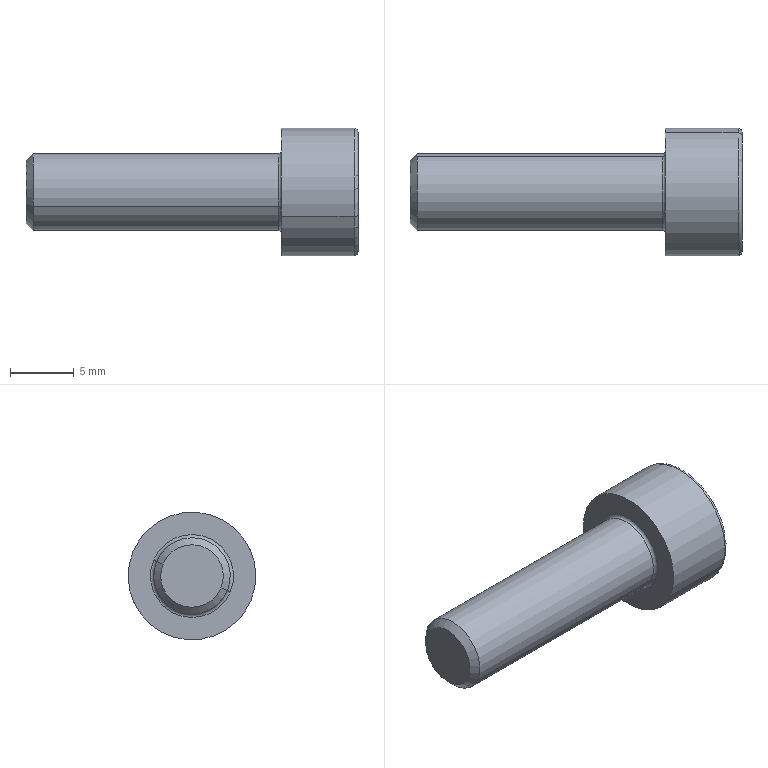Component | SolidWorks | bearing dan rumahan assembly-1_socket head cap screw_iso_M6x20-2 | 1 solid | 27 faces | box 26 x 10 x 10 mm | volume 957 mm3 | plane 15 | cone 4 | torus 4 | cylinder 4 | commonest cylinder face diameters 10 x2 6 x2
STEP:
#1=CARTESIAN_POINT('',(1.931,-4.331,3.445));
#2=VERTEX_POINT('',#1);
#3=CARTESIAN_POINT('',(1.988,-4.238,3.483));
#4=VERTEX_POINT('',#3);
#5=CARTESIAN_POINT('',(1.988,-4.238,3.483));
#6=DIRECTION('',(0.5,0.8004,0.3307));
#7=VECTOR('',#6,39.37);
#8=LINE('',#5,#7);
#9=EDGE_CURVE('',#2,#4,#8,.T.);
#10=ORIENTED_EDGE('',*,*,#9,.F.);
#11=CARTESIAN_POINT('',(1.988,-4.423,3.407));
#12=VERTEX_POINT('',#11);
#13=CARTESIAN_POINT('',(1.988,-4.423,3.407));
#14=DIRECTION('',(0.5,-0.8004,-0.3307));
#15=VECTOR('',#14,39.37);
#16=LINE('',#13,#15);
#17=EDGE_CURVE('',#2,#12,#16,.T.);
#18=ORIENTED_EDGE('',*,*,#17,.T.);
#19=CARTESIAN_POINT('',(1.988,-4.344,3.346));
#20=VERTEX_POINT('',#19);
#21=CARTESIAN_POINT('',(1.988,-4.331,3.445));
#22=DIRECTION('',(1.,0.,0.));
#23=DIRECTION('',(0.,0.9242,0.3818));
#24=AXIS2_PLACEMENT_3D('',#21,#22,#23);
#25=CIRCLE('',#24,0.0998);
#26=EDGE_CURVE('',#12,#20,#25,.T.);
#27=ORIENTED_EDGE('',*,*,#26,.T.);
#28=CARTESIAN_POINT('',(1.988,-4.252,3.384));
#29=VERTEX_POINT('',#28);
#30=CARTESIAN_POINT('',(1.988,-4.331,3.445));
#31=DIRECTION('',(1.,0.,0.));
#32=DIRECTION('',(0.,0.9242,0.3818));
#33=AXIS2_PLACEMENT_3D('',#30,#31,#32);
#34=CIRCLE('',#33,0.0998);
#35=EDGE_CURVE('',#20,#29,#34,.T.);
#36=ORIENTED_EDGE('',*,*,#35,.T.);
#37=CARTESIAN_POINT('',(1.988,-4.331,3.445));
#38=DIRECTION('',(1.,0.,0.));
#39=DIRECTION('',(0.,0.9242,0.3818));
#40=AXIS2_PLACEMENT_3D('',#37,#38,#39);
#41=CIRCLE('',#40,0.0998);
#42=EDGE_CURVE('',#29,#4,#41,.T.);
#43=ORIENTED_EDGE('',*,*,#42,.T.);
#44=EDGE_LOOP('',(#10,#18,#27,#36,#43));
#45=FACE_OUTER_BOUND('',#44,.T.);
#46=CARTESIAN_POINT('',(1.988,-4.331,3.445));
#47=DIRECTION('',(1.,0.,0.));
#48=DIRECTION('',(0.,0.9242,0.3818));
#49=AXIS2_PLACEMENT_3D('',#46,#47,#48);
#50=CONICAL_SURFACE('',#49,0.0998,1.047);
#51=ADVANCED_FACE('',(#45),#50,.F.);
#52=CARTESIAN_POINT('',(2.094,-4.513,3.37));
#53=VERTEX_POINT('',#52);
#54=CARTESIAN_POINT('',(2.094,-4.149,3.52));
#55=VERTEX_POINT('',#54);
#56=CARTESIAN_POINT('',(2.094,-4.331,3.445));
#57=DIRECTION('',(-1.,0.,0.));
#58=DIRECTION('',(0.,0.9242,0.3818));
#59=AXIS2_PLACEMENT_3D('',#56,#57,#58);
#60=CIRCLE('',#59,0.1969);
#61=EDGE_CURVE('',#53,#55,#60,.T.);
#62=ORIENTED_EDGE('',*,*,#61,.F.);
#63=CARTESIAN_POINT('',(2.106,-4.502,3.374));
#64=VERTEX_POINT('',#63);
#65=CARTESIAN_POINT('',(2.094,-4.502,3.374));
#66=DIRECTION('',(0.,-0.3818,0.9242));
#67=DIRECTION('',(0.,-0.9242,-0.3818));
#68=AXIS2_PLACEMENT_3D('',#65,#66,#67);
#69=CIRCLE('',#68,0.01181);
#70=EDGE_CURVE('',#53,#64,#69,.T.);
#71=ORIENTED_EDGE('',*,*,#70,.T.);
#72=CARTESIAN_POINT('',(2.106,-4.16,3.516));
#73=VERTEX_POINT('',#72);
#74=CARTESIAN_POINT('',(2.106,-4.331,3.445));
#75=DIRECTION('',(1.,0.,0.));
#76=DIRECTION('',(0.,0.9242,0.3818));
#77=AXIS2_PLACEMENT_3D('',#74,#75,#76);
#78=CIRCLE('',#77,0.185);
#79=EDGE_CURVE('',#73,#64,#78,.T.);
#80=ORIENTED_EDGE('',*,*,#79,.F.);
#81=CARTESIAN_POINT('',(2.094,-4.16,3.516));
#82=DIRECTION('',(0.,0.3818,-0.9242));
#83=DIRECTION('',(0.,0.9242,0.3818));
#84=AXIS2_PLACEMENT_3D('',#81,#82,#83);
#85=CIRCLE('',#84,0.01181);
#86=EDGE_CURVE('',#55,#73,#85,.T.);
#87=ORIENTED_EDGE('',*,*,#86,.F.);
#88=EDGE_LOOP('',(#62,#71,#80,#87));
#89=FACE_OUTER_BOUND('',#88,.T.);
#90=CARTESIAN_POINT('',(2.094,-4.331,3.445));
#91=DIRECTION('',(1.,0.,0.));
#92=DIRECTION('',(0.,0.9242,0.3818));
#93=AXIS2_PLACEMENT_3D('',#90,#91,#92);
#94=TOROIDAL_SURFACE('',#93,0.185,0.01181);
#95=ADVANCED_FACE('',(#89),#94,.T.);
#96=CARTESIAN_POINT('',(1.86,-4.222,3.49));
#97=VERTEX_POINT('',#96);
#98=CARTESIAN_POINT('',(1.86,-4.44,3.4));
#99=VERTEX_POINT('',#98);
#100=CARTESIAN_POINT('',(1.86,-4.331,3.445));
#101=DIRECTION('',(-1.,0.,0.));
#102=DIRECTION('',(0.,-0.9242,-0.3818));
#103=AXIS2_PLACEMENT_3D('',#100,#101,#102);
#104=CIRCLE('',#103,0.1181);
#105=EDGE_CURVE('',#97,#99,#104,.T.);
#106=ORIENTED_EDGE('',*,*,#105,.F.);
#107=CARTESIAN_POINT('',(1.87,-4.212,3.494));
#108=VERTEX_POINT('',#107);
#109=CARTESIAN_POINT('',(1.86,-4.212,3.494));
#110=DIRECTION('',(0.,-0.3818,0.9242));
#111=DIRECTION('',(0.,-0.9242,-0.3818));
#112=AXIS2_PLACEMENT_3D('',#109,#110,#111);
#113=CIRCLE('',#112,0.009843);
#114=EDGE_CURVE('',#97,#108,#113,.T.);
#115=ORIENTED_EDGE('',*,*,#114,.T.);
#116=CARTESIAN_POINT('',(1.87,-4.449,3.396));
#117=VERTEX_POINT('',#116);
#118=CARTESIAN_POINT('',(1.87,-4.331,3.445));
#119=DIRECTION('',(1.,0.,0.));
#120=DIRECTION('',(0.,-0.9242,-0.3818));
#121=AXIS2_PLACEMENT_3D('',#118,#119,#120);
#122=CIRCLE('',#121,0.128);
#123=EDGE_CURVE('',#117,#108,#122,.T.);
#124=ORIENTED_EDGE('',*,*,#123,.F.);
#125=CARTESIAN_POINT('',(1.86,-4.449,3.396));
#126=DIRECTION('',(0.,0.3818,-0.9242));
#127=DIRECTION('',(0.,0.9242,0.3818));
#128=AXIS2_PLACEMENT_3D('',#125,#126,#127);
#129=CIRCLE('',#128,0.009843);
#130=EDGE_CURVE('',#99,#117,#129,.T.);
#131=ORIENTED_EDGE('',*,*,#130,.F.);
#132=EDGE_LOOP('',(#106,#115,#124,#131));
#133=FACE_OUTER_BOUND('',#132,.T.);
#134=CARTESIAN_POINT('',(1.86,-4.331,3.445));
#135=DIRECTION('',(-1.,0.,0.));
#136=DIRECTION('',(0.,-0.9242,-0.3818));
#137=AXIS2_PLACEMENT_3D('',#134,#135,#136);
#138=TOROIDAL_SURFACE('',#137,0.128,0.009843);
#139=ADVANCED_FACE('',(#133),#138,.F.);
#140=CARTESIAN_POINT('',(1.87,-4.149,3.52));
#141=VERTEX_POINT('',#140);
#142=CARTESIAN_POINT('',(1.87,-4.513,3.37));
#143=VERTEX_POINT('',#142);
#144=CARTESIAN_POINT('',(1.87,-4.331,3.445));
#145=DIRECTION('',(1.,0.,0.));
#146=DIRECTION('',(0.,0.9242,0.3818));
#147=AXIS2_PLACEMENT_3D('',#144,#145,#146);
#148=CIRCLE('',#147,0.1969);
#149=EDGE_CURVE('',#141,#143,#148,.T.);
#150=ORIENTED_EDGE('',*,*,#149,.T.);
#151=CARTESIAN_POINT('',(3.356,-4.513,3.37));
#152=DIRECTION('',(1.,0.,0.));
#153=VECTOR('',#152,39.37);
#154=LINE('',#151,#153);
#155=EDGE_CURVE('',#143,#53,#154,.T.);
#156=ORIENTED_EDGE('',*,*,#155,.T.);
#157=ORIENTED_EDGE('',*,*,#61,.T.);
#158=CARTESIAN_POINT('',(3.356,-4.149,3.52));
#159=DIRECTION('',(1.,0.,0.));
#160=VECTOR('',#159,39.37);
#161=LINE('',#158,#160);
#162=EDGE_CURVE('',#141,#55,#161,.T.);
#163=ORIENTED_EDGE('',*,*,#162,.F.);
#164=EDGE_LOOP('',(#150,#156,#157,#163));
#165=FACE_OUTER_BOUND('',#164,.T.);
#166=CARTESIAN_POINT('',(3.356,-4.331,3.445));
#167=DIRECTION('',(1.,0.,0.));
#168=DIRECTION('',(0.,0.9242,0.3818));
#169=AXIS2_PLACEMENT_3D('',#166,#167,#168);
#170=CYLINDRICAL_SURFACE('',#169,0.1969);
#171=ADVANCED_FACE('',(#165),#170,.T.);
#172=CARTESIAN_POINT('',(1.104,-4.222,3.49));
#173=VERTEX_POINT('',#172);
#174=CARTESIAN_POINT('',(1.104,-4.44,3.4));
#175=VERTEX_POINT('',#174);
#176=CARTESIAN_POINT('',(1.104,-4.331,3.445));
#177=DIRECTION('',(1.,0.,0.));
#178=DIRECTION('',(0.,0.9242,0.3818));
#179=AXIS2_PLACEMENT_3D('',#176,#177,#178);
#180=CIRCLE('',#179,0.1181);
#181=EDGE_CURVE('',#173,#175,#180,.T.);
#182=ORIENTED_EDGE('',*,*,#181,.T.);
#183=CARTESIAN_POINT('',(3.356,-4.44,3.4));
#184=DIRECTION('',(1.,0.,0.));
#185=VECTOR('',#184,39.37);
#186=LINE('',#183,#185);
#187=EDGE_CURVE('',#175,#99,#186,.T.);
#188=ORIENTED_EDGE('',*,*,#187,.T.);
#189=CARTESIAN_POINT('',(1.86,-4.331,3.445));
#190=DIRECTION('',(-1.,0.,0.));
#191=DIRECTION('',(0.,-0.9242,-0.3818));
#192=AXIS2_PLACEMENT_3D('',#189,#190,#191);
#193=CIRCLE('',#192,0.1181);
#194=EDGE_CURVE('',#99,#97,#193,.T.);
#195=ORIENTED_EDGE('',*,*,#194,.T.);
#196=CARTESIAN_POINT('',(3.356,-4.222,3.49));
#197=DIRECTION('',(1.,0.,0.));
#198=VECTOR('',#197,39.37);
#199=LINE('',#196,#198);
#200=EDGE_CURVE('',#173,#97,#199,.T.);
#201=ORIENTED_EDGE('',*,*,#200,.F.);
#202=EDGE_LOOP('',(#182,#188,#195,#201));
#203=FACE_OUTER_BOUND('',#202,.T.);
#204=CARTESIAN_POINT('',(3.356,-4.331,3.445));
#205=DIRECTION('',(1.,0.,0.));
#206=DIRECTION('',(0.,0.9242,0.3818));
#207=AXIS2_PLACEMENT_3D('',#204,#205,#206);
#208=CYLINDRICAL_SURFACE('',#207,0.1181);
#209=ADVANCED_FACE('',(#203),#208,.T.);
#210=CARTESIAN_POINT('',(1.083,-4.242,3.482));
#211=VERTEX_POINT('',#210);
#212=CARTESIAN_POINT('',(1.083,-4.42,3.408));
#213=VERTEX_POINT('',#212);
#214=CARTESIAN_POINT('',(1.083,-4.331,3.445));
#215=DIRECTION('',(1.,0.,0.));
#216=DIRECTION('',(0.,0.9242,0.3818));
#217=AXIS2_PLACEMENT_3D('',#214,#215,#216);
#218=CIRCLE('',#217,0.0965);
#219=EDGE_CURVE('',#211,#213,#218,.T.);
#220=ORIENTED_EDGE('',*,*,#219,.T.);
#221=CARTESIAN_POINT('',(1.083,-4.42,3.408));
#222=DIRECTION('',(0.7071,-0.6535,-0.27));
#223=VECTOR('',#222,39.37);
#224=LINE('',#221,#223);
#225=EDGE_CURVE('',#213,#175,#224,.T.);
#226=ORIENTED_EDGE('',*,*,#225,.T.);
#227=ORIENTED_EDGE('',*,*,#181,.F.);
#228=CARTESIAN_POINT('',(1.083,-4.242,3.482));
#229=DIRECTION('',(0.7071,0.6535,0.27));
#230=VECTOR('',#229,39.37);
#231=LINE('',#228,#230);
#232=EDGE_CURVE('',#211,#173,#231,.T.);
#233=ORIENTED_EDGE('',*,*,#232,.F.);
#234=EDGE_LOOP('',(#220,#226,#227,#233));
#235=FACE_OUTER_BOUND('',#234,.T.);
#236=CARTESIAN_POINT('',(1.083,-4.331,3.445));
#237=DIRECTION('',(1.,0.,0.));
#238=DIRECTION('',(0.,0.9242,0.3818));
#239=AXIS2_PLACEMENT_3D('',#236,#237,#238);
#240=CONICAL_SURFACE('',#239,0.0965,0.7854);
#241=ADVANCED_FACE('',(#235),#240,.T.);
#242=CARTESIAN_POINT('',(2.106,-4.375,3.551));
#243=VERTEX_POINT('',#242);
#244=CARTESIAN_POINT('',(2.106,-4.26,3.536));
#245=VERTEX_POINT('',#244);
#246=CARTESIAN_POINT('',(2.106,-4.375,3.551));
#247=DIRECTION('',(0.,0.9913,-0.1314));
#248=VECTOR('',#247,39.37);
#249=LINE('',#246,#248);
#250=EDGE_CURVE('',#243,#245,#249,.T.);
#251=ORIENTED_EDGE('',*,*,#250,.T.);
#252=CARTESIAN_POINT('',(2.106,-4.216,3.43));
#253=VERTEX_POINT('',#252);
#254=CARTESIAN_POINT('',(2.106,-4.216,3.43));
#255=DIRECTION('',(0.,-0.3818,0.9242));
#256=VECTOR('',#255,39.37);
#257=LINE('',#254,#256);
#258=EDGE_CURVE('',#253,#245,#257,.T.);
#259=ORIENTED_EDGE('',*,*,#258,.F.);
#260=CARTESIAN_POINT('',(2.106,-4.287,3.338));
#261=VERTEX_POINT('',#260);
#262=CARTESIAN_POINT('',(2.106,-4.216,3.43));
#263=DIRECTION('',(0.,-0.6095,-0.7928));
#264=VECTOR('',#263,39.37);
#265=LINE('',#262,#264);
#266=EDGE_CURVE('',#253,#261,#265,.T.);
#267=ORIENTED_EDGE('',*,*,#266,.T.);
#268=CARTESIAN_POINT('',(2.106,-4.401,3.354));
#269=VERTEX_POINT('',#268);
#270=CARTESIAN_POINT('',(2.106,-4.287,3.338));
#271=DIRECTION('',(0.,-0.9913,0.1314));
#272=VECTOR('',#271,39.37);
#273=LINE('',#270,#272);
#274=EDGE_CURVE('',#261,#269,#273,.T.);
#275=ORIENTED_EDGE('',*,*,#274,.T.);
#276=CARTESIAN_POINT('',(2.106,-4.445,3.46));
#277=VERTEX_POINT('',#276);
#278=CARTESIAN_POINT('',(2.106,-4.445,3.46));
#279=DIRECTION('',(0.,0.3818,-0.9242));
#280=VECTOR('',#279,39.37);
#281=LINE('',#278,#280);
#282=EDGE_CURVE('',#277,#269,#281,.T.);
#283=ORIENTED_EDGE('',*,*,#282,.F.);
#284=CARTESIAN_POINT('',(2.106,-4.375,3.551));
#285=DIRECTION('',(0.,-0.6095,-0.7928));
#286=VECTOR('',#285,39.37);
#287=LINE('',#284,#286);
#288=EDGE_CURVE('',#243,#277,#287,.T.);
#289=ORIENTED_EDGE('',*,*,#288,.F.);
#290=EDGE_LOOP('',(#251,#259,#267,#275,#283,#289));
#291=FACE_BOUND('',#290,.T.);
#292=ORIENTED_EDGE('',*,*,#79,.T.);
#293=CARTESIAN_POINT('',(2.106,-4.331,3.445));
#294=DIRECTION('',(1.,0.,0.));
#295=DIRECTION('',(0.,0.9242,0.3818));
#296=AXIS2_PLACEMENT_3D('',#293,#294,#295);
#297=CIRCLE('',#296,0.185);
#298=EDGE_CURVE('',#64,#73,#297,.T.);
#299=ORIENTED_EDGE('',*,*,#298,.T.);
#300=EDGE_LOOP('',(#292,#299));
#301=FACE_OUTER_BOUND('',#300,.T.);
#302=CARTESIAN_POINT('',(2.106,-4.331,3.445));
#303=DIRECTION('',(1.,0.,0.));
#304=DIRECTION('',(0.,0.9242,0.3818));
#305=AXIS2_PLACEMENT_3D('',#302,#303,#304);
#306=PLANE('',#305);
#307=ADVANCED_FACE('',(#291,#301),#306,.T.);
#308=ORIENTED_EDGE('',*,*,#219,.F.);
#309=CARTESIAN_POINT('',(1.083,-4.331,3.445));
#310=DIRECTION('',(1.,0.,0.));
#311=DIRECTION('',(0.,0.9242,0.3818));
#312=AXIS2_PLACEMENT_3D('',#309,#310,#311);
#313=CIRCLE('',#312,0.0965);
#314=EDGE_CURVE('',#213,#211,#313,.T.);
#315=ORIENTED_EDGE('',*,*,#314,.F.);
#316=EDGE_LOOP('',(#308,#315));
#317=FACE_OUTER_BOUND('',#316,.T.);
#318=CARTESIAN_POINT('',(1.083,-4.368,3.534));
#319=DIRECTION('',(-1.,0.,0.));
#320=DIRECTION('',(0.,-0.9242,-0.3818));
#321=AXIS2_PLACEMENT_3D('',#318,#319,#320);
#322=PLANE('',#321);
#323=ADVANCED_FACE('',(#317),#322,.T.);
#324=ORIENTED_EDGE('',*,*,#225,.F.);
#325=ORIENTED_EDGE('',*,*,#314,.T.);
#326=ORIENTED_EDGE('',*,*,#232,.T.);
#327=CARTESIAN_POINT('',(1.104,-4.331,3.445));
#328=DIRECTION('',(1.,0.,0.));
#329=DIRECTION('',(0.,0.9242,0.3818));
#330=AXIS2_PLACEMENT_3D('',#327,#328,#329);
#331=CIRCLE('',#330,0.1181);
#332=EDGE_CURVE('',#175,#173,#331,.T.);
#333=ORIENTED_EDGE('',*,*,#332,.F.);
#334=EDGE_LOOP('',(#324,#325,#326,#333));
#335=FACE_OUTER_BOUND('',#334,.T.);
#336=CARTESIAN_POINT('',(1.083,-4.331,3.445));
#337=DIRECTION('',(1.,0.,0.));
#338=DIRECTION('',(0.,0.9242,0.3818));
#339=AXIS2_PLACEMENT_3D('',#336,#337,#338);
#340=CONICAL_SURFACE('',#339,0.0965,0.7854);
#341=ADVANCED_FACE('',(#335),#340,.T.);
#342=ORIENTED_EDGE('',*,*,#187,.F.);
#343=ORIENTED_EDGE('',*,*,#332,.T.);
#344=ORIENTED_EDGE('',*,*,#200,.T.);
#345=ORIENTED_EDGE('',*,*,#105,.T.);
#346=EDGE_LOOP('',(#342,#343,#344,#345));
#347=FACE_OUTER_BOUND('',#346,.T.);
#348=CARTESIAN_POINT('',(3.356,-4.331,3.445));
#349=DIRECTION('',(1.,0.,0.));
#350=DIRECTION('',(0.,0.9242,0.3818));
#351=AXIS2_PLACEMENT_3D('',#348,#349,#350);
#352=CYLINDRICAL_SURFACE('',#351,0.1181);
#353=ADVANCED_FACE('',(#347),#352,.T.);
#354=ORIENTED_EDGE('',*,*,#123,.T.);
#355=CARTESIAN_POINT('',(1.87,-4.331,3.445));
#356=DIRECTION('',(1.,0.,0.));
#357=DIRECTION('',(0.,-0.9242,-0.3818));
#358=AXIS2_PLACEMENT_3D('',#355,#356,#357);
#359=CIRCLE('',#358,0.128);
#360=EDGE_CURVE('',#108,#117,#359,.T.);
#361=ORIENTED_EDGE('',*,*,#360,.T.);
#362=EDGE_LOOP('',(#354,#361));
#363=FACE_BOUND('',#362,.T.);
#364=ORIENTED_EDGE('',*,*,#149,.F.);
#365=CARTESIAN_POINT('',(1.87,-4.331,3.445));
#366=DIRECTION('',(1.,0.,0.));
#367=DIRECTION('',(0.,0.9242,0.3818));
#368=AXIS2_PLACEMENT_3D('',#365,#366,#367);
#369=CIRCLE('',#368,0.1969);
#370=EDGE_CURVE('',#143,#141,#369,.T.);
#371=ORIENTED_EDGE('',*,*,#370,.F.);
#372=EDGE_LOOP('',(#364,#371));
#373=FACE_OUTER_BOUND('',#372,.T.);
#374=CARTESIAN_POINT('',(1.87,-4.406,3.627));
#375=DIRECTION('',(-1.,0.,0.));
#376=DIRECTION('',(0.,-0.9242,-0.3818));
#377=AXIS2_PLACEMENT_3D('',#374,#375,#376);
#378=PLANE('',#377);
#379=ADVANCED_FACE('',(#363,#373),#378,.T.);
#380=ORIENTED_EDGE('',*,*,#155,.F.);
#381=ORIENTED_EDGE('',*,*,#370,.T.);
#382=ORIENTED_EDGE('',*,*,#162,.T.);
#383=CARTESIAN_POINT('',(2.094,-4.331,3.445));
#384=DIRECTION('',(-1.,0.,0.));
#385=DIRECTION('',(0.,0.9242,0.3818));
#386=AXIS2_PLACEMENT_3D('',#383,#384,#385);
#387=CIRCLE('',#386,0.1969);
#388=EDGE_CURVE('',#55,#53,#387,.T.);
#389=ORIENTED_EDGE('',*,*,#388,.T.);
#390=EDGE_LOOP('',(#380,#381,#382,#389));
#391=FACE_OUTER_BOUND('',#390,.T.);
#392=CARTESIAN_POINT('',(3.356,-4.331,3.445));
#393=DIRECTION('',(1.,0.,0.));
#394=DIRECTION('',(0.,0.9242,0.3818));
#395=AXIS2_PLACEMENT_3D('',#392,#393,#394);
#396=CYLINDRICAL_SURFACE('',#395,0.1969);
#397=ADVANCED_FACE('',(#391),#396,.T.);
#398=ORIENTED_EDGE('',*,*,#114,.F.);
#399=ORIENTED_EDGE('',*,*,#194,.F.);
#400=ORIENTED_EDGE('',*,*,#130,.T.);
#401=ORIENTED_EDGE('',*,*,#360,.F.);
#402=EDGE_LOOP('',(#398,#399,#400,#401));
#403=FACE_OUTER_BOUND('',#402,.T.);
#404=CARTESIAN_POINT('',(1.86,-4.331,3.445));
#405=DIRECTION('',(-1.,0.,0.));
#406=DIRECTION('',(0.,-0.9242,-0.3818));
#407=AXIS2_PLACEMENT_3D('',#404,#405,#406);
#408=TOROIDAL_SURFACE('',#407,0.128,0.009843);
#409=ADVANCED_FACE('',(#403),#408,.F.);
#410=ORIENTED_EDGE('',*,*,#70,.F.);
#411=ORIENTED_EDGE('',*,*,#388,.F.);
#412=ORIENTED_EDGE('',*,*,#86,.T.);
#413=ORIENTED_EDGE('',*,*,#298,.F.);
#414=EDGE_LOOP('',(#410,#411,#412,#413));
#415=FACE_OUTER_BOUND('',#414,.T.);
#416=CARTESIAN_POINT('',(2.094,-4.331,3.445));
#417=DIRECTION('',(1.,0.,0.));
#418=DIRECTION('',(0.,0.9242,0.3818));
#419=AXIS2_PLACEMENT_3D('',#416,#417,#418);
#420=TOROIDAL_SURFACE('',#419,0.185,0.01181);
#421=ADVANCED_FACE('',(#415),#420,.T.);
#422=ORIENTED_EDGE('',*,*,#250,.F.);
#423=CARTESIAN_POINT('',(1.988,-4.375,3.551));
#424=VERTEX_POINT('',#423);
#425=CARTESIAN_POINT('',(1.988,-4.375,3.551));
#426=DIRECTION('',(1.,0.,0.));
#427=VECTOR('',#426,39.37);
#428=LINE('',#425,#427);
#429=EDGE_CURVE('',#424,#243,#428,.T.);
#430=ORIENTED_EDGE('',*,*,#429,.F.);
#431=CARTESIAN_POINT('',(1.988,-4.318,3.544));
#432=VERTEX_POINT('',#431);
#433=CARTESIAN_POINT('',(1.988,-4.375,3.551));
#434=DIRECTION('',(0.,0.9913,-0.1314));
#435=VECTOR('',#434,39.37);
#436=LINE('',#433,#435);
#437=EDGE_CURVE('',#424,#432,#436,.T.);
#438=ORIENTED_EDGE('',*,*,#437,.T.);
#439=CARTESIAN_POINT('',(1.988,-4.26,3.536));
#440=VERTEX_POINT('',#439);
#441=CARTESIAN_POINT('',(1.988,-4.375,3.551));
#442=DIRECTION('',(0.,0.9913,-0.1314));
#443=VECTOR('',#442,39.37);
#444=LINE('',#441,#443);
#445=EDGE_CURVE('',#432,#440,#444,.T.);
#446=ORIENTED_EDGE('',*,*,#445,.T.);
#447=CARTESIAN_POINT('',(1.988,-4.26,3.536));
#448=DIRECTION('',(1.,0.,0.));
#449=VECTOR('',#448,39.37);
#450=LINE('',#447,#449);
#451=EDGE_CURVE('',#440,#245,#450,.T.);
#452=ORIENTED_EDGE('',*,*,#451,.T.);
#453=EDGE_LOOP('',(#422,#430,#438,#446,#452));
#454=FACE_OUTER_BOUND('',#453,.T.);
#455=CARTESIAN_POINT('',(1.988,-4.375,3.551));
#456=DIRECTION('',(0.,-0.1314,-0.9913));
#457=DIRECTION('',(0.,-0.9913,0.1314));
#458=AXIS2_PLACEMENT_3D('',#455,#456,#457);
#459=PLANE('',#458);
#460=ADVANCED_FACE('',(#454),#459,.T.);
#461=ORIENTED_EDGE('',*,*,#258,.T.);
#462=ORIENTED_EDGE('',*,*,#451,.F.);
#463=CARTESIAN_POINT('',(1.988,-4.216,3.43));
#464=DIRECTION('',(0.,-0.3818,0.9242));
#465=VECTOR('',#464,39.37);
#466=LINE('',#463,#465);
#467=EDGE_CURVE('',#4,#440,#466,.T.);
#468=ORIENTED_EDGE('',*,*,#467,.F.);
#469=CARTESIAN_POINT('',(1.988,-4.216,3.43));
#470=VERTEX_POINT('',#469);
#471=CARTESIAN_POINT('',(1.988,-4.216,3.43));
#472=DIRECTION('',(0.,-0.3818,0.9242));
#473=VECTOR('',#472,39.37);
#474=LINE('',#471,#473);
#475=EDGE_CURVE('',#470,#4,#474,.T.);
#476=ORIENTED_EDGE('',*,*,#475,.F.);
#477=CARTESIAN_POINT('',(1.988,-4.216,3.43));
#478=DIRECTION('',(1.,0.,0.));
#479=VECTOR('',#478,39.37);
#480=LINE('',#477,#479);
#481=EDGE_CURVE('',#470,#253,#480,.T.);
#482=ORIENTED_EDGE('',*,*,#481,.T.);
#483=EDGE_LOOP('',(#461,#462,#468,#476,#482));
#484=FACE_OUTER_BOUND('',#483,.T.);
#485=CARTESIAN_POINT('',(1.988,-4.216,3.43));
#486=DIRECTION('',(0.,0.9242,0.3818));
#487=DIRECTION('',(0.,0.3818,-0.9242));
#488=AXIS2_PLACEMENT_3D('',#485,#486,#487);
#489=PLANE('',#488);
#490=ADVANCED_FACE('',(#484),#489,.F.);
#491=ORIENTED_EDGE('',*,*,#266,.F.);
#492=ORIENTED_EDGE('',*,*,#481,.F.);
#493=CARTESIAN_POINT('',(1.988,-4.216,3.43));
#494=DIRECTION('',(0.,-0.6095,-0.7928));
#495=VECTOR('',#494,39.37);
#496=LINE('',#493,#495);
#497=EDGE_CURVE('',#470,#29,#496,.T.);
#498=ORIENTED_EDGE('',*,*,#497,.T.);
#499=CARTESIAN_POINT('',(1.988,-4.287,3.338));
#500=VERTEX_POINT('',#499);
#501=CARTESIAN_POINT('',(1.988,-4.216,3.43));
#502=DIRECTION('',(0.,-0.6095,-0.7928));
#503=VECTOR('',#502,39.37);
#504=LINE('',#501,#503);
#505=EDGE_CURVE('',#29,#500,#504,.T.);
#506=ORIENTED_EDGE('',*,*,#505,.T.);
#507=CARTESIAN_POINT('',(1.988,-4.287,3.338));
#508=DIRECTION('',(1.,0.,0.));
#509=VECTOR('',#508,39.37);
#510=LINE('',#507,#509);
#511=EDGE_CURVE('',#500,#261,#510,.T.);
#512=ORIENTED_EDGE('',*,*,#511,.T.);
#513=EDGE_LOOP('',(#491,#492,#498,#506,#512));
#514=FACE_OUTER_BOUND('',#513,.T.);
#515=CARTESIAN_POINT('',(1.988,-4.216,3.43));
#516=DIRECTION('',(0.,-0.7928,0.6095));
#517=DIRECTION('',(0.,0.6095,0.7928));
#518=AXIS2_PLACEMENT_3D('',#515,#516,#517);
#519=PLANE('',#518);
#520=ADVANCED_FACE('',(#514),#519,.T.);
#521=ORIENTED_EDGE('',*,*,#274,.F.);
#522=ORIENTED_EDGE('',*,*,#511,.F.);
#523=CARTESIAN_POINT('',(1.988,-4.287,3.338));
#524=DIRECTION('',(0.,-0.9913,0.1314));
#525=VECTOR('',#524,39.37);
#526=LINE('',#523,#525);
#527=EDGE_CURVE('',#500,#20,#526,.T.);
#528=ORIENTED_EDGE('',*,*,#527,.T.);
#529=CARTESIAN_POINT('',(1.988,-4.401,3.354));
#530=VERTEX_POINT('',#529);
#531=CARTESIAN_POINT('',(1.988,-4.287,3.338));
#532=DIRECTION('',(0.,-0.9913,0.1314));
#533=VECTOR('',#532,39.37);
#534=LINE('',#531,#533);
#535=EDGE_CURVE('',#20,#530,#534,.T.);
#536=ORIENTED_EDGE('',*,*,#535,.T.);
#537=CARTESIAN_POINT('',(1.988,-4.401,3.354));
#538=DIRECTION('',(1.,0.,0.));
#539=VECTOR('',#538,39.37);
#540=LINE('',#537,#539);
#541=EDGE_CURVE('',#530,#269,#540,.T.);
#542=ORIENTED_EDGE('',*,*,#541,.T.);
#543=EDGE_LOOP('',(#521,#522,#528,#536,#542));
#544=FACE_OUTER_BOUND('',#543,.T.);
#545=CARTESIAN_POINT('',(1.988,-4.287,3.338));
#546=DIRECTION('',(0.,0.1314,0.9913));
#547=DIRECTION('',(0.,0.9913,-0.1314));
#548=AXIS2_PLACEMENT_3D('',#545,#546,#547);
#549=PLANE('',#548);
#550=ADVANCED_FACE('',(#544),#549,.T.);
#551=ORIENTED_EDGE('',*,*,#282,.T.);
#552=ORIENTED_EDGE('',*,*,#541,.F.);
#553=CARTESIAN_POINT('',(1.988,-4.445,3.46));
#554=DIRECTION('',(0.,0.3818,-0.9242));
#555=VECTOR('',#554,39.37);
#556=LINE('',#553,#555);
#557=EDGE_CURVE('',#12,#530,#556,.T.);
#558=ORIENTED_EDGE('',*,*,#557,.F.);
#559=CARTESIAN_POINT('',(1.988,-4.445,3.46));
#560=VERTEX_POINT('',#559);
#561=CARTESIAN_POINT('',(1.988,-4.445,3.46));
#562=DIRECTION('',(0.,0.3818,-0.9242));
#563=VECTOR('',#562,39.37);
#564=LINE('',#561,#563);
#565=EDGE_CURVE('',#560,#12,#564,.T.);
#566=ORIENTED_EDGE('',*,*,#565,.F.);
#567=CARTESIAN_POINT('',(1.988,-4.445,3.46));
#568=DIRECTION('',(1.,0.,0.));
#569=VECTOR('',#568,39.37);
#570=LINE('',#567,#569);
#571=EDGE_CURVE('',#560,#277,#570,.T.);
#572=ORIENTED_EDGE('',*,*,#571,.T.);
#573=EDGE_LOOP('',(#551,#552,#558,#566,#572));
#574=FACE_OUTER_BOUND('',#573,.T.);
#575=CARTESIAN_POINT('',(1.988,-4.445,3.46));
#576=DIRECTION('',(0.,-0.9242,-0.3818));
#577=DIRECTION('',(0.,-0.3818,0.9242));
#578=AXIS2_PLACEMENT_3D('',#575,#576,#577);
#579=PLANE('',#578);
#580=ADVANCED_FACE('',(#574),#579,.F.);
#581=ORIENTED_EDGE('',*,*,#288,.T.);
#582=ORIENTED_EDGE('',*,*,#571,.F.);
#583=CARTESIAN_POINT('',(1.988,-4.41,3.506));
#584=VERTEX_POINT('',#583);
#585=CARTESIAN_POINT('',(1.988,-4.375,3.551));
#586=DIRECTION('',(0.,-0.6095,-0.7928));
#587=VECTOR('',#586,39.37);
#588=LINE('',#585,#587);
#589=EDGE_CURVE('',#584,#560,#588,.T.);
#590=ORIENTED_EDGE('',*,*,#589,.F.);
#591=CARTESIAN_POINT('',(1.988,-4.375,3.551));
#592=DIRECTION('',(0.,-0.6095,-0.7928));
#593=VECTOR('',#592,39.37);
#594=LINE('',#591,#593);
#595=EDGE_CURVE('',#424,#584,#594,.T.);
#596=ORIENTED_EDGE('',*,*,#595,.F.);
#597=ORIENTED_EDGE('',*,*,#429,.T.);
#598=EDGE_LOOP('',(#581,#582,#590,#596,#597));
#599=FACE_OUTER_BOUND('',#598,.T.);
#600=CARTESIAN_POINT('',(1.988,-4.375,3.551));
#601=DIRECTION('',(0.,-0.7928,0.6095));
#602=DIRECTION('',(0.,0.6095,0.7928));
#603=AXIS2_PLACEMENT_3D('',#600,#601,#602);
#604=PLANE('',#603);
#605=ADVANCED_FACE('',(#599),#604,.F.);
#606=ORIENTED_EDGE('',*,*,#557,.T.);
#607=ORIENTED_EDGE('',*,*,#535,.F.);
#608=ORIENTED_EDGE('',*,*,#26,.F.);
#609=EDGE_LOOP('',(#606,#607,#608));
#610=FACE_OUTER_BOUND('',#609,.T.);
#611=CARTESIAN_POINT('',(1.988,-4.375,3.551));
#612=DIRECTION('',(-1.,0.,0.));
#613=DIRECTION('',(0.,-0.9242,-0.3818));
#614=AXIS2_PLACEMENT_3D('',#611,#612,#613);
#615=PLANE('',#614);
#616=ADVANCED_FACE('',(#610),#615,.F.);
#617=ORIENTED_EDGE('',*,*,#527,.F.);
#618=ORIENTED_EDGE('',*,*,#505,.F.);
#619=ORIENTED_EDGE('',*,*,#35,.F.);
#620=EDGE_LOOP('',(#617,#618,#619));
#621=FACE_OUTER_BOUND('',#620,.T.);
#622=CARTESIAN_POINT('',(1.988,-4.375,3.551));
#623=DIRECTION('',(-1.,0.,0.));
#624=DIRECTION('',(0.,-0.9242,-0.3818));
#625=AXIS2_PLACEMENT_3D('',#622,#623,#624);
#626=PLANE('',#625);
#627=ADVANCED_FACE('',(#621),#626,.F.);
#628=ORIENTED_EDGE('',*,*,#497,.F.);
#629=ORIENTED_EDGE('',*,*,#475,.T.);
#630=ORIENTED_EDGE('',*,*,#42,.F.);
#631=EDGE_LOOP('',(#628,#629,#630));
#632=FACE_OUTER_BOUND('',#631,.T.);
#633=CARTESIAN_POINT('',(1.988,-4.375,3.551));
#634=DIRECTION('',(-1.,0.,0.));
#635=DIRECTION('',(0.,-0.9242,-0.3818));
#636=AXIS2_PLACEMENT_3D('',#633,#634,#635);
#637=PLANE('',#636);
#638=ADVANCED_FACE('',(#632),#637,.F.);
#639=ORIENTED_EDGE('',*,*,#467,.T.);
#640=ORIENTED_EDGE('',*,*,#445,.F.);
#641=CARTESIAN_POINT('',(1.988,-4.331,3.445));
#642=DIRECTION('',(1.,0.,0.));
#643=DIRECTION('',(0.,0.9242,0.3818));
#644=AXIS2_PLACEMENT_3D('',#641,#642,#643);
#645=CIRCLE('',#644,0.0998);
#646=EDGE_CURVE('',#4,#432,#645,.T.);
#647=ORIENTED_EDGE('',*,*,#646,.F.);
#648=EDGE_LOOP('',(#639,#640,#647));
#649=FACE_OUTER_BOUND('',#648,.T.);
#650=CARTESIAN_POINT('',(1.988,-4.375,3.551));
#651=DIRECTION('',(-1.,0.,0.));
#652=DIRECTION('',(0.,-0.9242,-0.3818));
#653=AXIS2_PLACEMENT_3D('',#650,#651,#652);
#654=PLANE('',#653);
#655=ADVANCED_FACE('',(#649),#654,.F.);
#656=ORIENTED_EDGE('',*,*,#437,.F.);
#657=ORIENTED_EDGE('',*,*,#595,.T.);
#658=CARTESIAN_POINT('',(1.988,-4.331,3.445));
#659=DIRECTION('',(1.,0.,0.));
#660=DIRECTION('',(0.,0.9242,0.3818));
#661=AXIS2_PLACEMENT_3D('',#658,#659,#660);
#662=CIRCLE('',#661,0.0998);
#663=EDGE_CURVE('',#432,#584,#662,.T.);
#664=ORIENTED_EDGE('',*,*,#663,.F.);
#665=EDGE_LOOP('',(#656,#657,#664));
#666=FACE_OUTER_BOUND('',#665,.T.);
#667=CARTESIAN_POINT('',(1.988,-4.375,3.551));
#668=DIRECTION('',(-1.,0.,0.));
#669=DIRECTION('',(0.,-0.9242,-0.3818));
#670=AXIS2_PLACEMENT_3D('',#667,#668,#669);
#671=PLANE('',#670);
#672=ADVANCED_FACE('',(#666),#671,.F.);
#673=ORIENTED_EDGE('',*,*,#589,.T.);
#674=ORIENTED_EDGE('',*,*,#565,.T.);
#675=CARTESIAN_POINT('',(1.988,-4.331,3.445));
#676=DIRECTION('',(1.,0.,0.));
#677=DIRECTION('',(0.,0.9242,0.3818));
#678=AXIS2_PLACEMENT_3D('',#675,#676,#677);
#679=CIRCLE('',#678,0.0998);
#680=EDGE_CURVE('',#584,#12,#679,.T.);
#681=ORIENTED_EDGE('',*,*,#680,.F.);
#682=EDGE_LOOP('',(#673,#674,#681));
#683=FACE_OUTER_BOUND('',#682,.T.);
#684=CARTESIAN_POINT('',(1.988,-4.375,3.551));
#685=DIRECTION('',(-1.,0.,0.));
#686=DIRECTION('',(0.,-0.9242,-0.3818));
#687=AXIS2_PLACEMENT_3D('',#684,#685,#686);
#688=PLANE('',#687);
#689=ADVANCED_FACE('',(#683),#688,.F.);
#690=ORIENTED_EDGE('',*,*,#17,.F.);
#691=ORIENTED_EDGE('',*,*,#9,.T.);
#692=ORIENTED_EDGE('',*,*,#646,.T.);
#693=ORIENTED_EDGE('',*,*,#663,.T.);
#694=ORIENTED_EDGE('',*,*,#680,.T.);
#695=EDGE_LOOP('',(#690,#691,#692,#693,#694));
#696=FACE_OUTER_BOUND('',#695,.T.);
#697=CARTESIAN_POINT('',(1.988,-4.331,3.445));
#698=DIRECTION('',(1.,0.,0.));
#699=DIRECTION('',(0.,0.9242,0.3818));
#700=AXIS2_PLACEMENT_3D('',#697,#698,#699);
#701=CONICAL_SURFACE('',#700,0.0998,1.047);
#702=ADVANCED_FACE('',(#696),#701,.F.);
#703=CLOSED_SHELL('',(#51,#95,#139,#171,#209,#241,#307,#323,#341,#353,#379,#397,#409,#421,#460,#490,#520,#550,#580,#605,#616,#627,#638,#655,#672,#689,#702));
#704=MANIFOLD_SOLID_BREP('',#703);
#705=CARTESIAN_POINT('',(0.,0.,0.));
#706=DIRECTION('',(0.,0.,1.));
#707=DIRECTION('',(1.,0.,0.));
#708=AXIS2_PLACEMENT_3D('',#705,#706,#707);
#709=(LENGTH_UNIT()NAMED_UNIT(*)SI_UNIT($,.METRE.));
#710=LENGTH_MEASURE_WITH_UNIT(LENGTH_MEASURE(0.0254),#709);
#711=DIMENSIONAL_EXPONENTS(1.,0.,0.,0.,0.,0.,0.);
#712=(CONVERSION_BASED_UNIT('',#710)LENGTH_UNIT()NAMED_UNIT(#711));
#713=UNCERTAINTY_MEASURE_WITH_UNIT(LENGTH_MEASURE(0.00001),#712,'','');
#714=(NAMED_UNIT(*)PLANE_ANGLE_UNIT()SI_UNIT($,.RADIAN.));
#715=(NAMED_UNIT(*)SI_UNIT($,.STERADIAN.)SOLID_ANGLE_UNIT());
#716=(GEOMETRIC_REPRESENTATION_CONTEXT(3)GLOBAL_UNCERTAINTY_ASSIGNED_CONTEXT((#713))GLOBAL_UNIT_ASSIGNED_CONTEXT((#712,#714,#715))REPRESENTATION_CONTEXT('',''));
#717=ADVANCED_BREP_SHAPE_REPRESENTATION('',(#704,#708),#716);
#718=COLOUR_RGB('',0.7922,0.8196,0.9333);
#719=FILL_AREA_STYLE_COLOUR('',#718);
#720=FILL_AREA_STYLE('',(#719));
#721=SURFACE_STYLE_FILL_AREA(#720);
#722=SURFACE_SIDE_STYLE('',(#721));
#723=SURFACE_STYLE_USAGE(.BOTH.,#722);
#724=PRESENTATION_STYLE_ASSIGNMENT((#723));
#725=STYLED_ITEM('',(#724),#704);
#726=(LENGTH_UNIT()NAMED_UNIT(*)SI_UNIT($,.METRE.));
#727=LENGTH_MEASURE_WITH_UNIT(LENGTH_MEASURE(0.0254),#726);
#728=DIMENSIONAL_EXPONENTS(1.,0.,0.,0.,0.,0.,0.);
#729=(CONVERSION_BASED_UNIT('',#727)LENGTH_UNIT()NAMED_UNIT(#728));
#730=UNCERTAINTY_MEASURE_WITH_UNIT(LENGTH_MEASURE(0.00001),#729,'','');
#731=(NAMED_UNIT(*)PLANE_ANGLE_UNIT()SI_UNIT($,.RADIAN.));
#732=(NAMED_UNIT(*)SI_UNIT($,.STERADIAN.)SOLID_ANGLE_UNIT());
#733=(GEOMETRIC_REPRESENTATION_CONTEXT(3)GLOBAL_UNCERTAINTY_ASSIGNED_CONTEXT((#730))GLOBAL_UNIT_ASSIGNED_CONTEXT((#729,#731,#732))REPRESENTATION_CONTEXT('',''));
#734=MECHANICAL_DESIGN_GEOMETRIC_PRESENTATION_REPRESENTATION('',(#725),#733);
#735=PRESENTATION_LAYER_ASSIGNMENT('','',(#725));